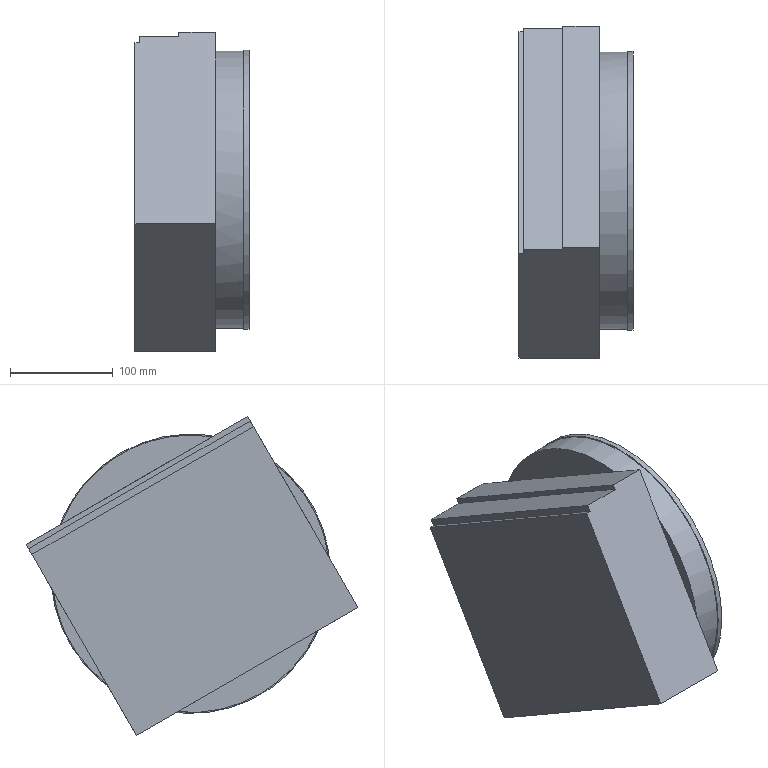Component | NX | SIM15_REV_SCHEIBE_AUFNAHME | 1 solid | 21 faces | volume 6007363 mm3 | plane 19 | cylinder 2 | commonest cylinder face diameters 270 x1 272 x1